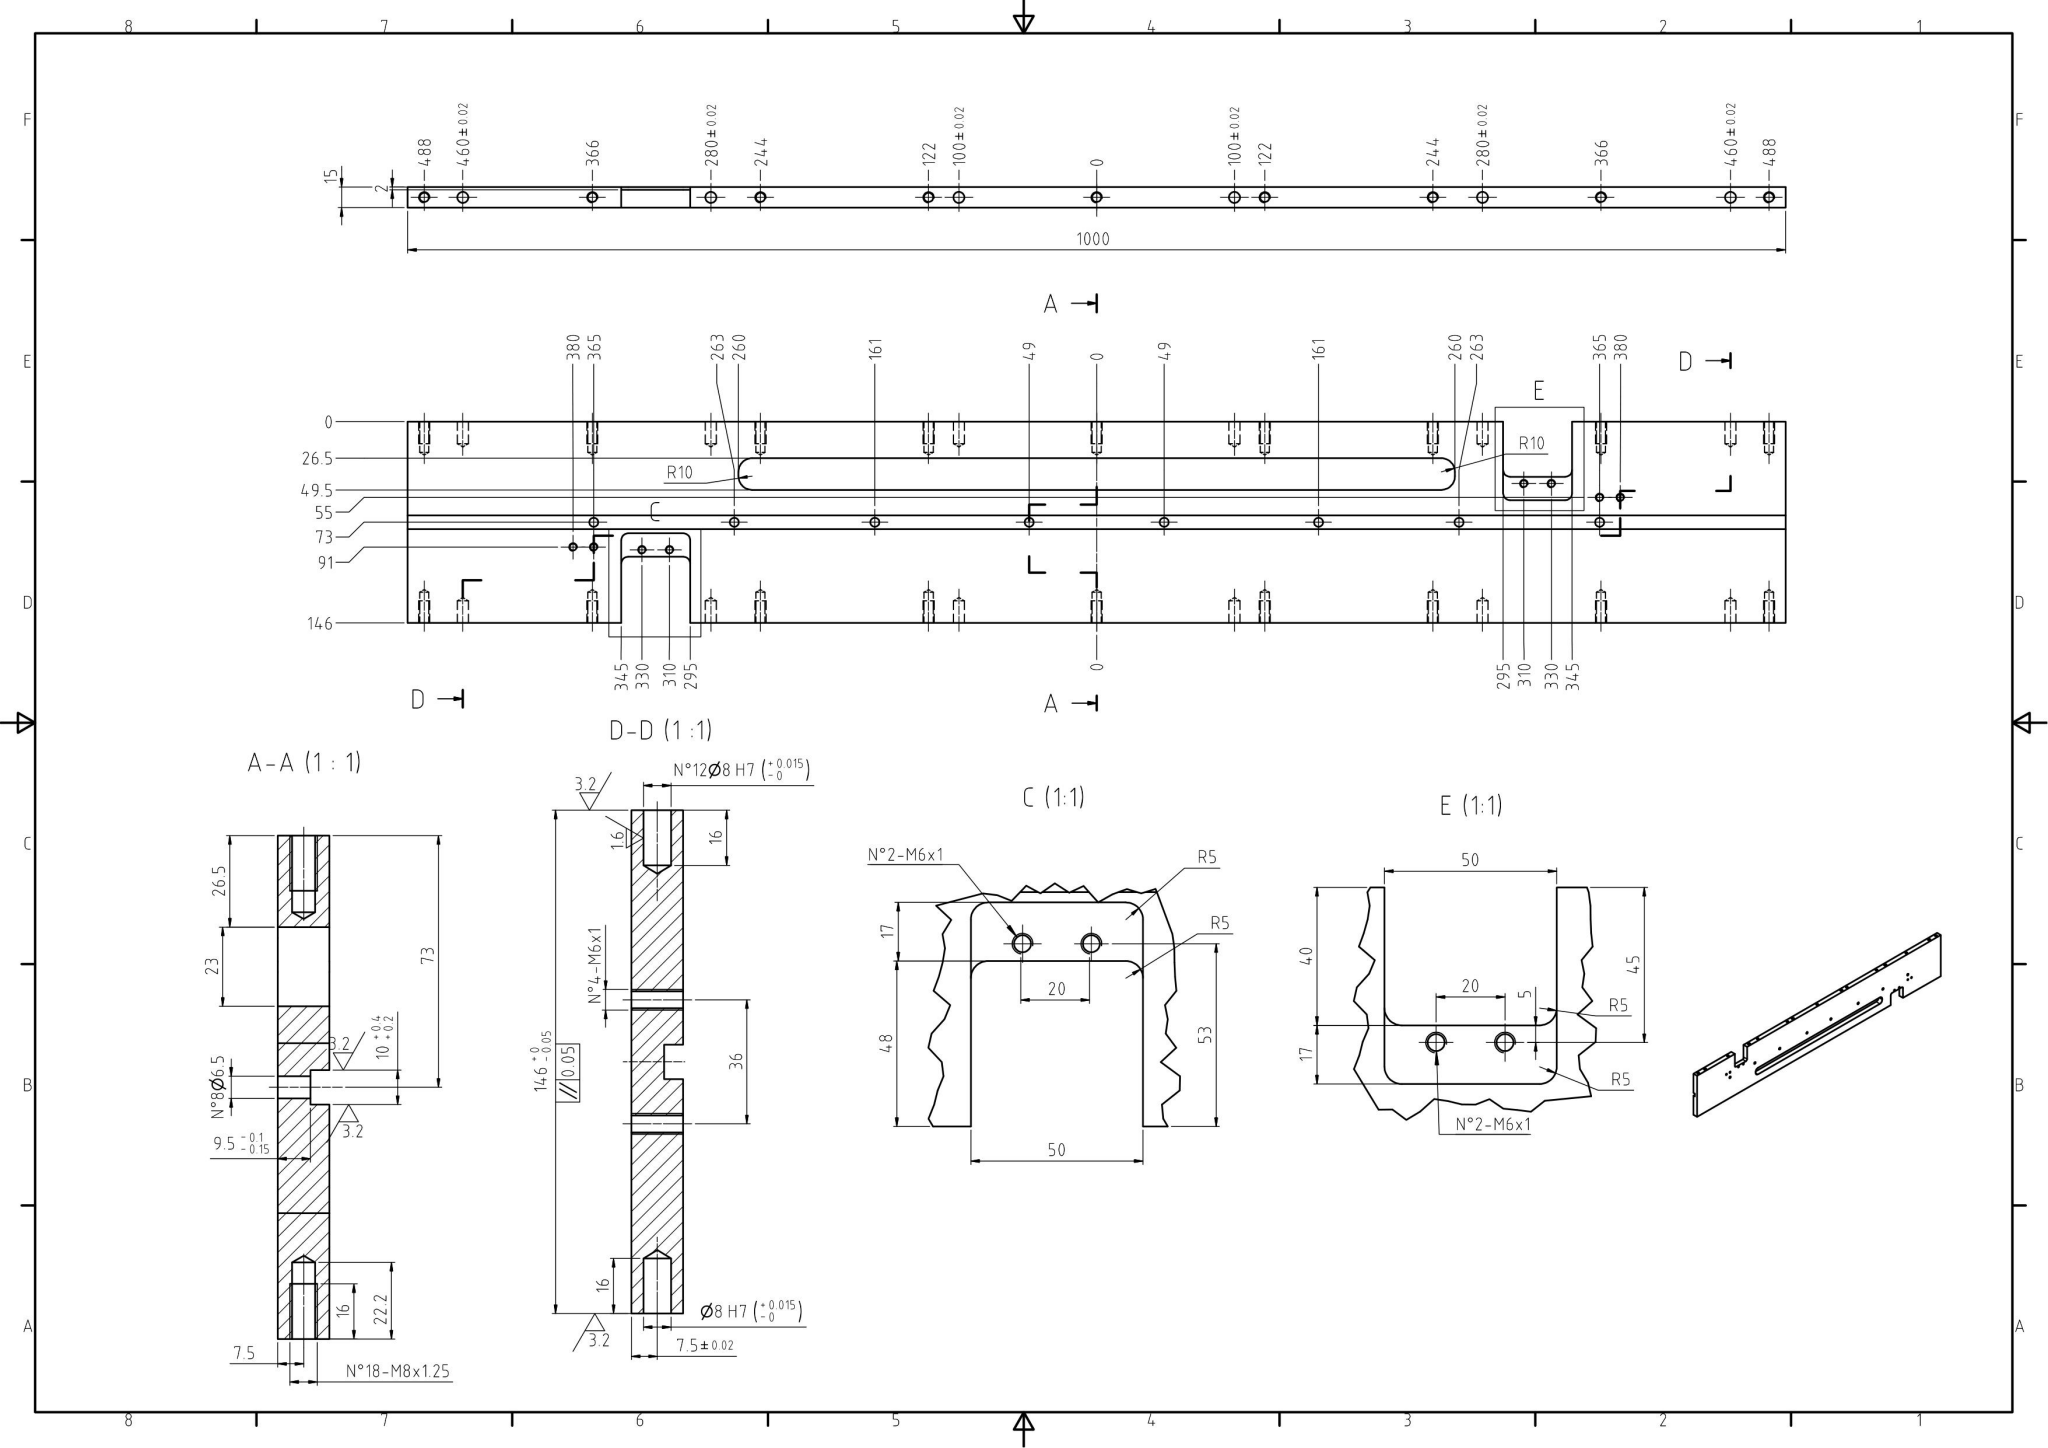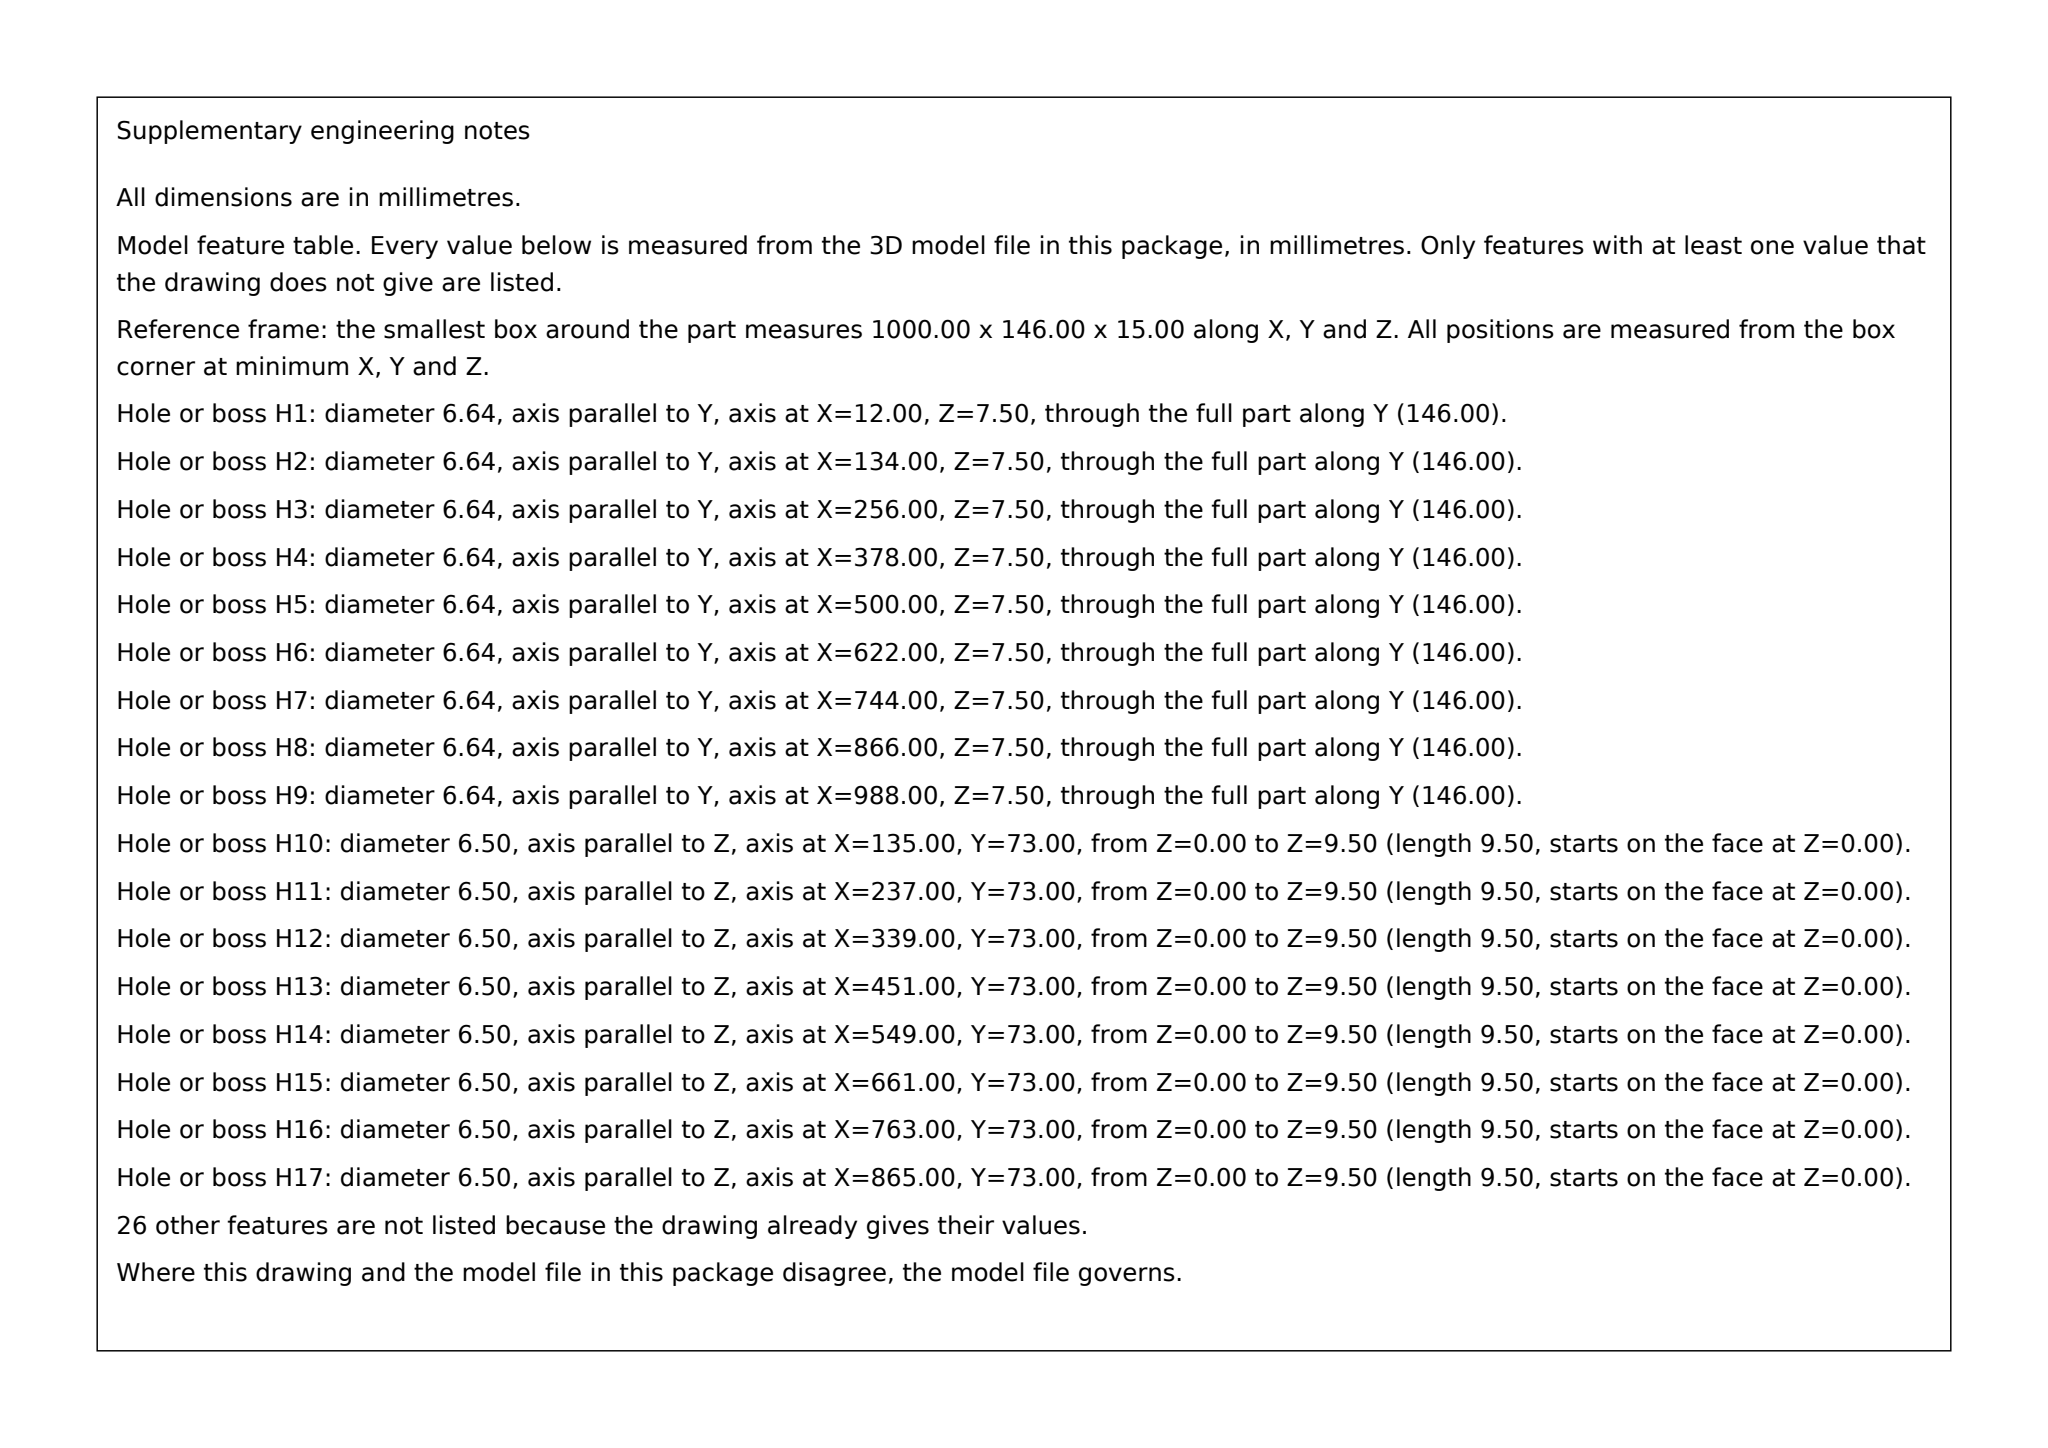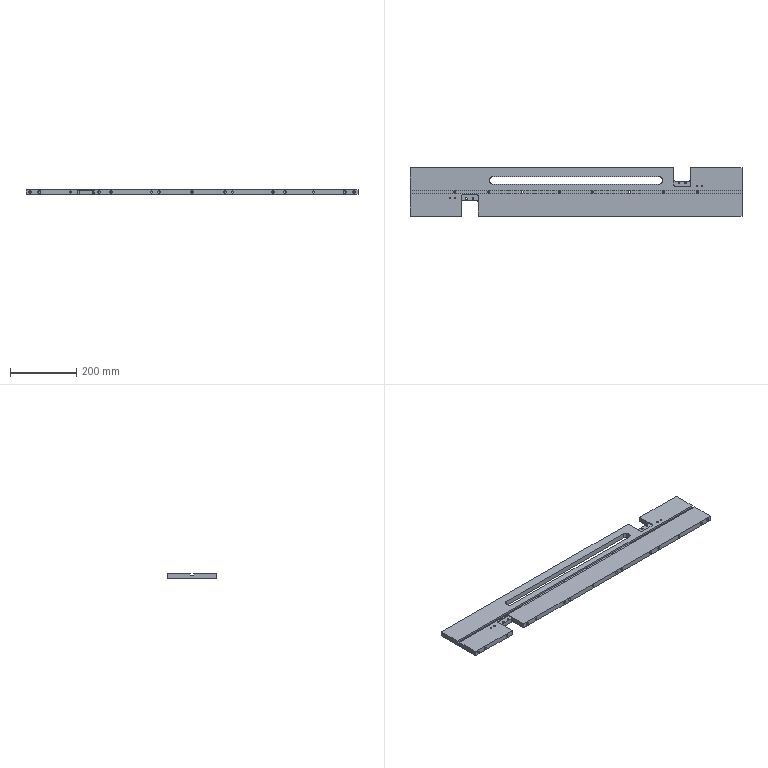Part | SolidWorks | mm | 1 solid | 202 faces | box 1000 x 146 x 15 mm | volume 1858744 mm3 | cylinder 116 | cone 60 | plane 26 | commonest cylinder face diameters 6.647 x36 8 x24 4.917 x16 10 x16 6.5 x16 20 x8